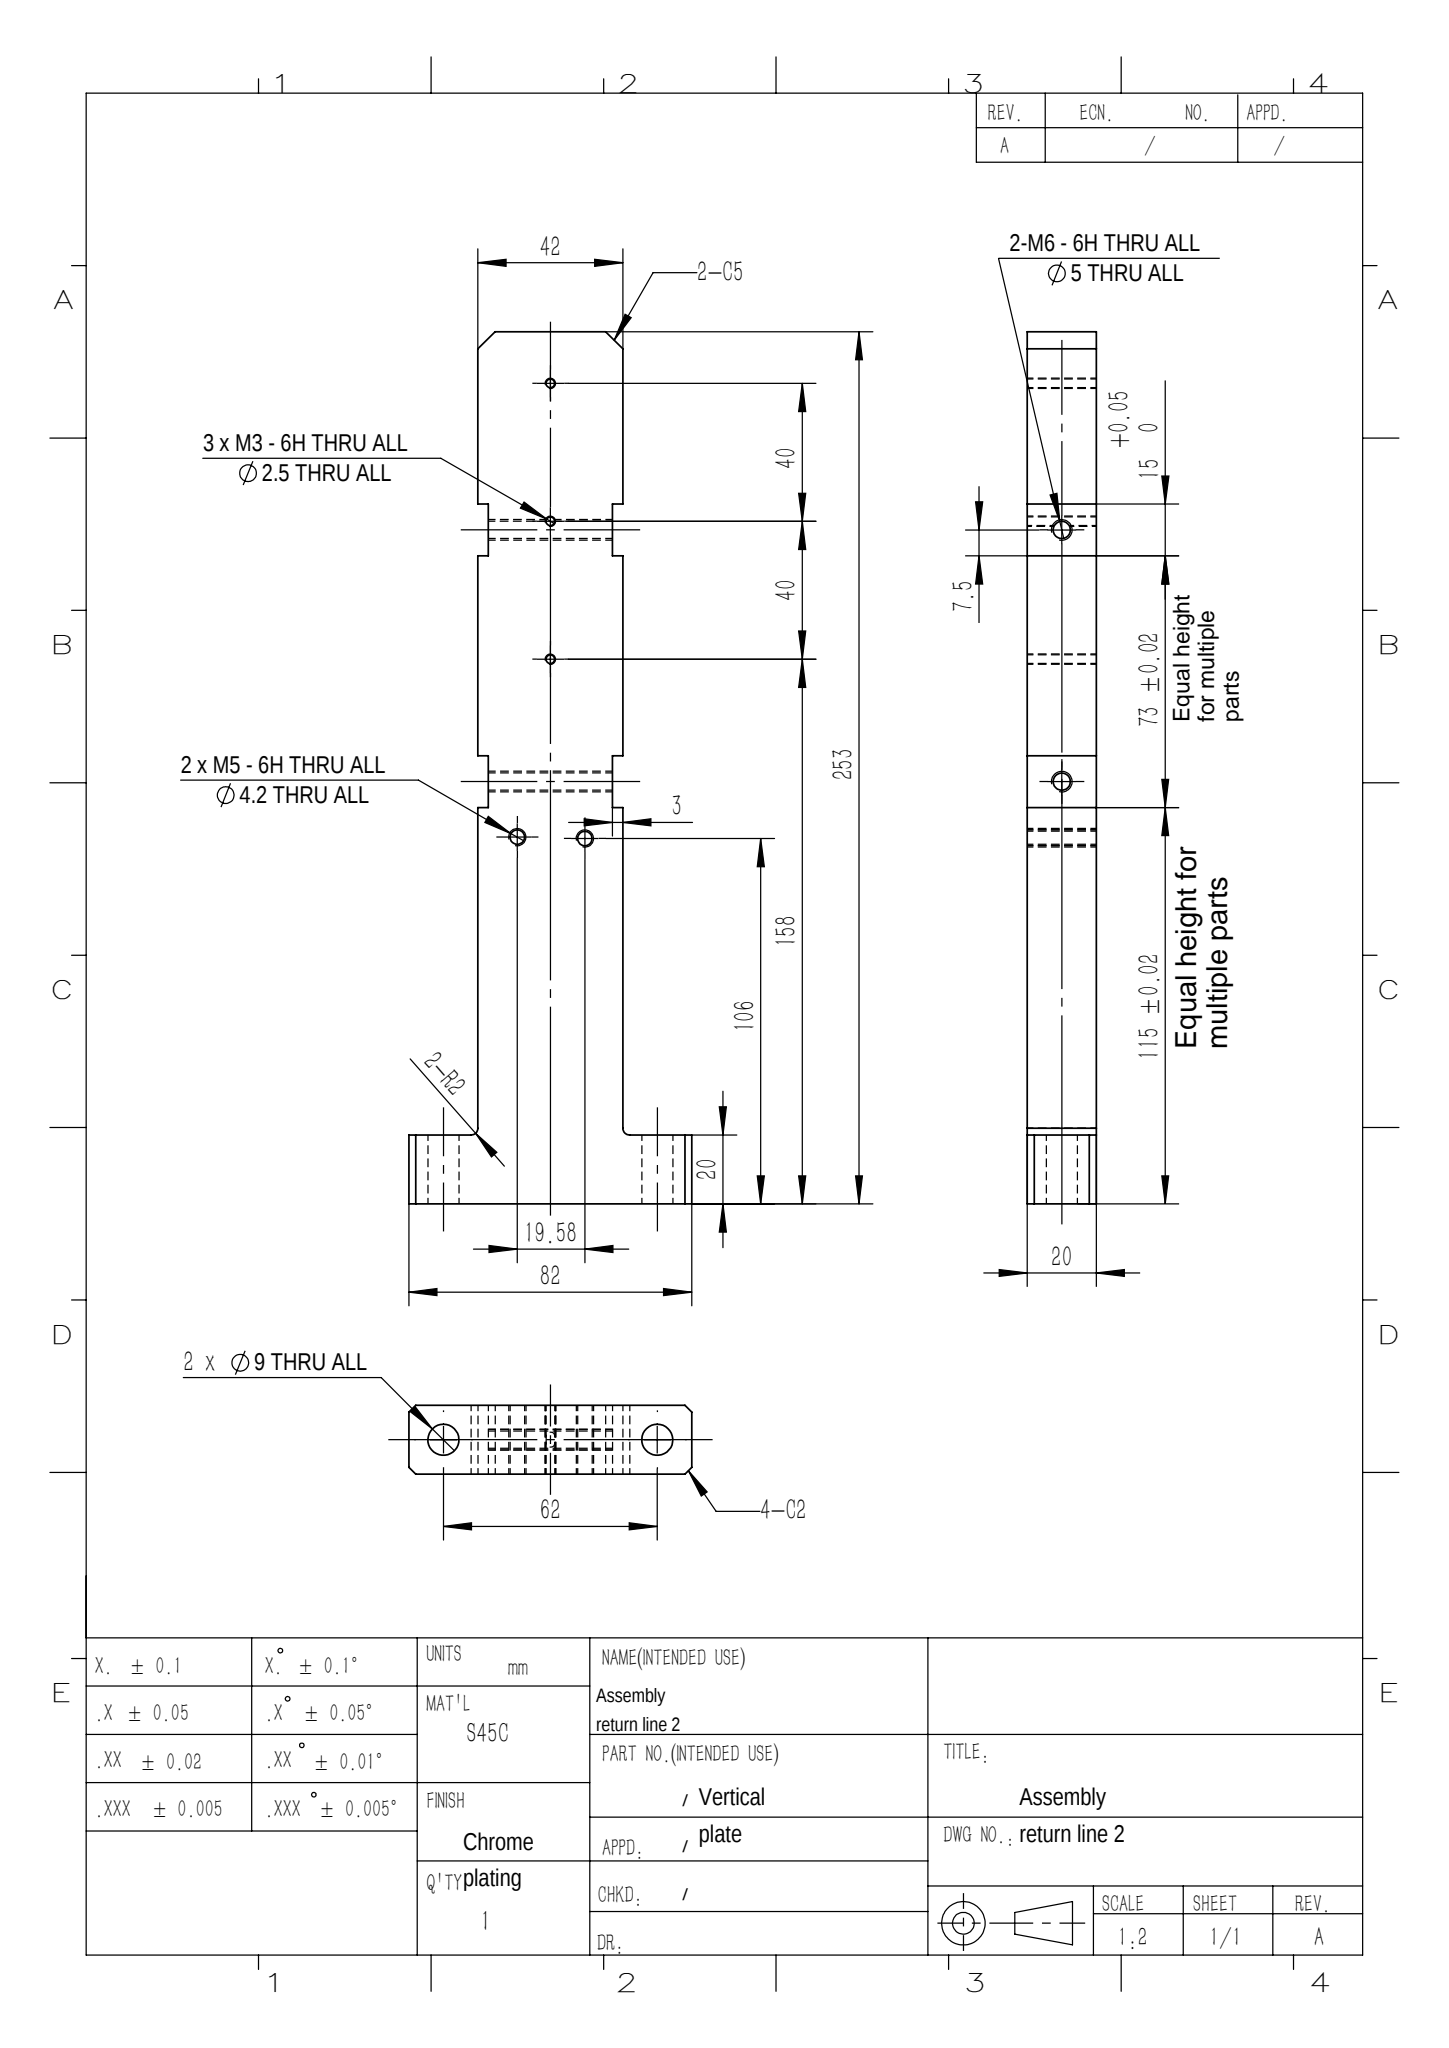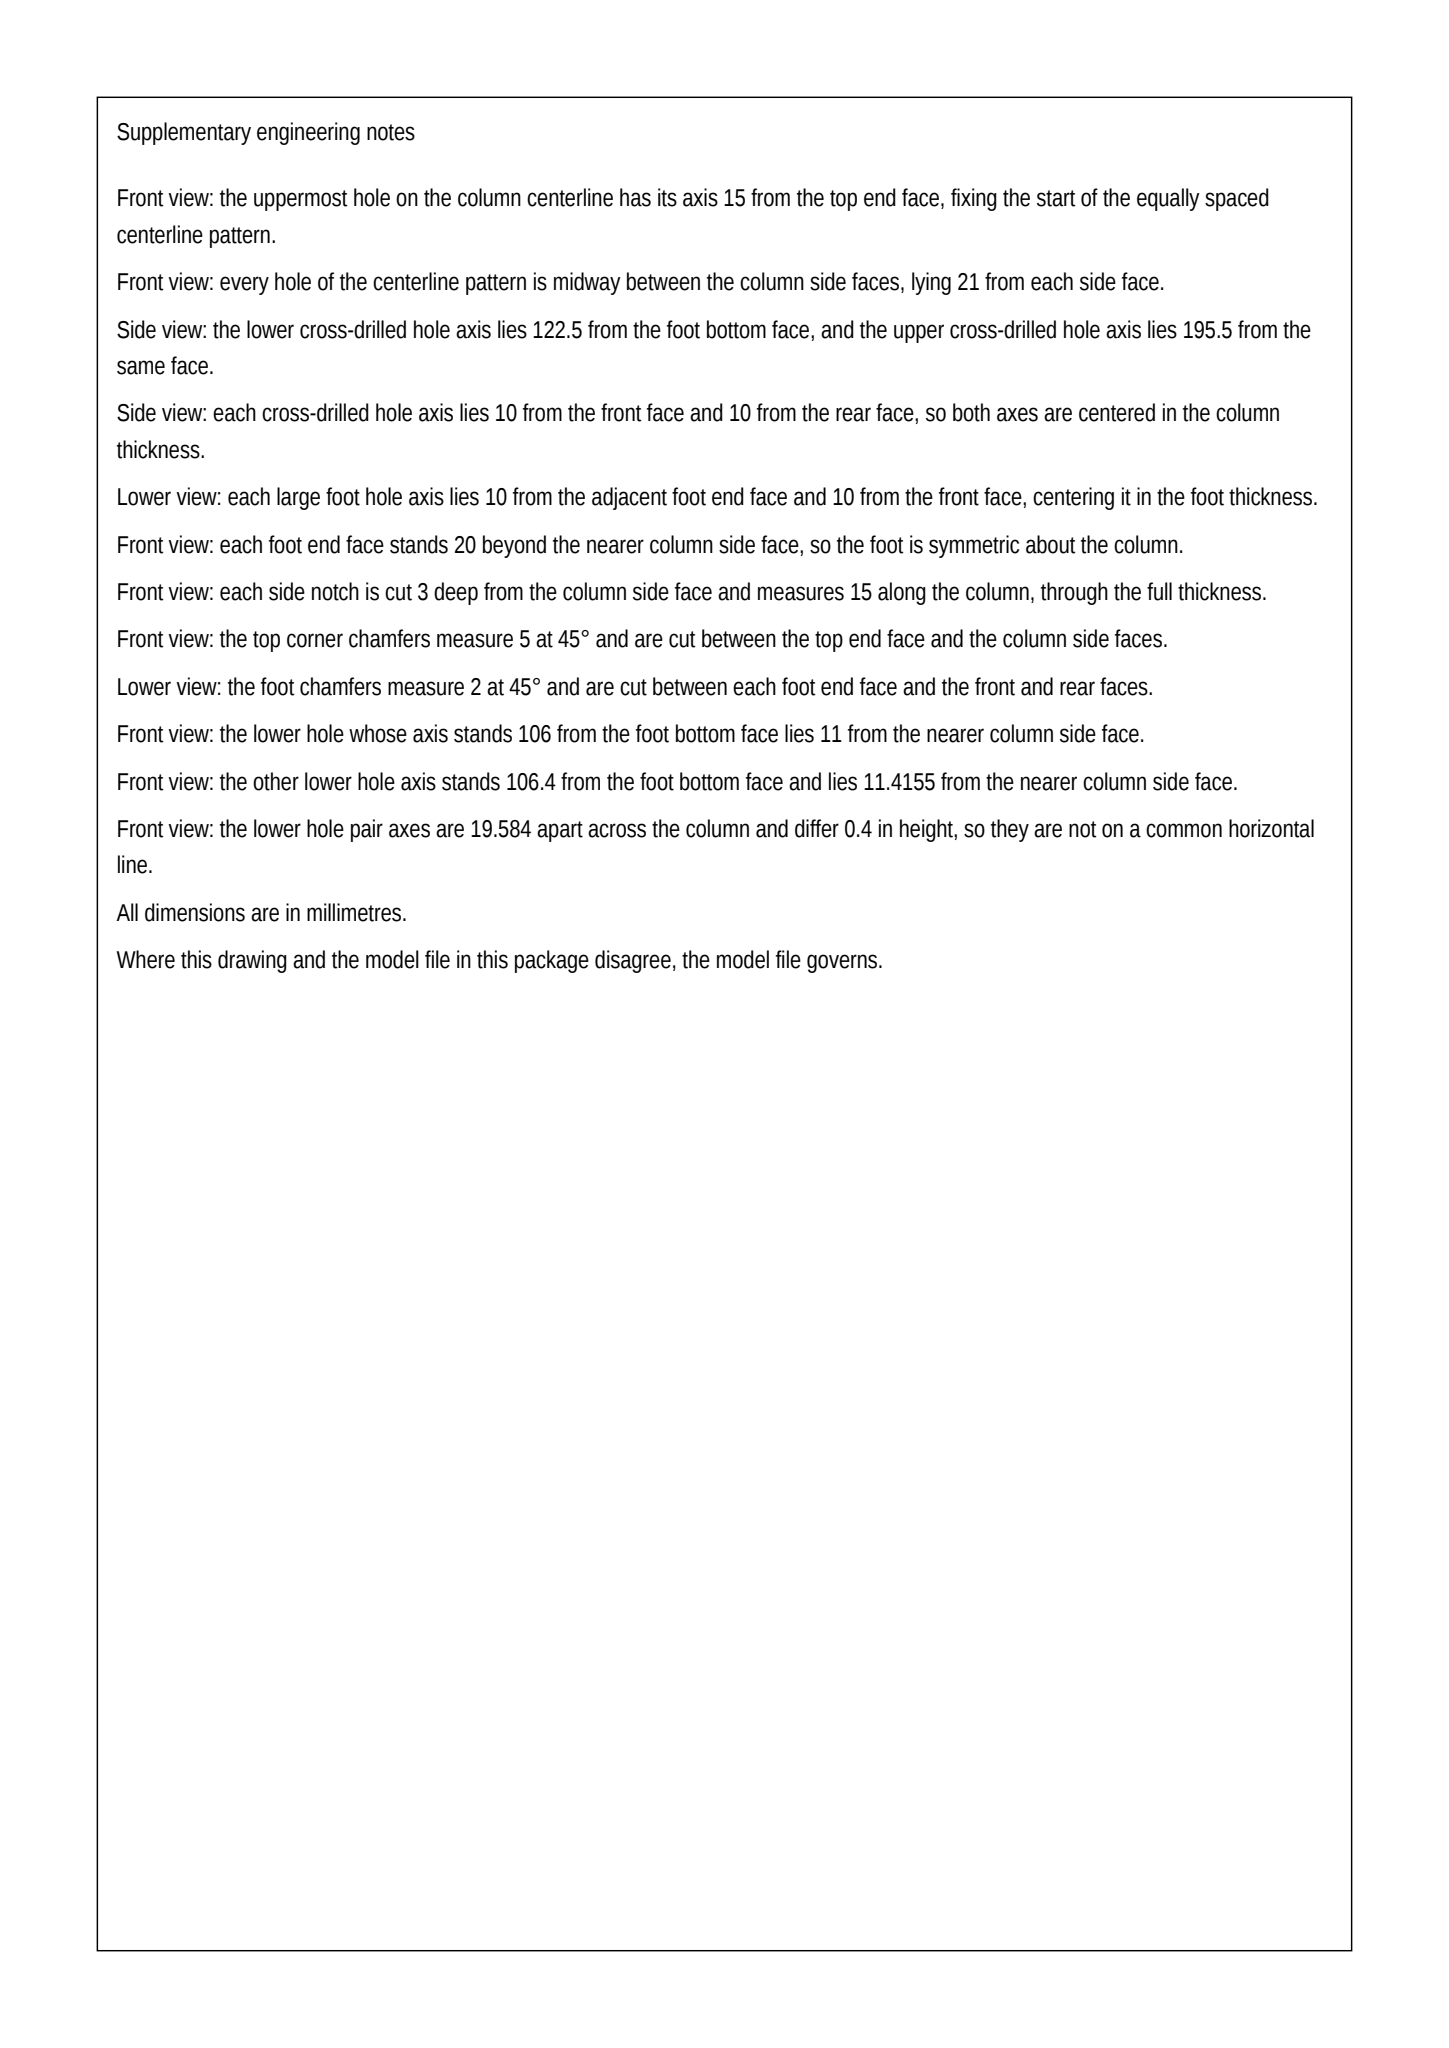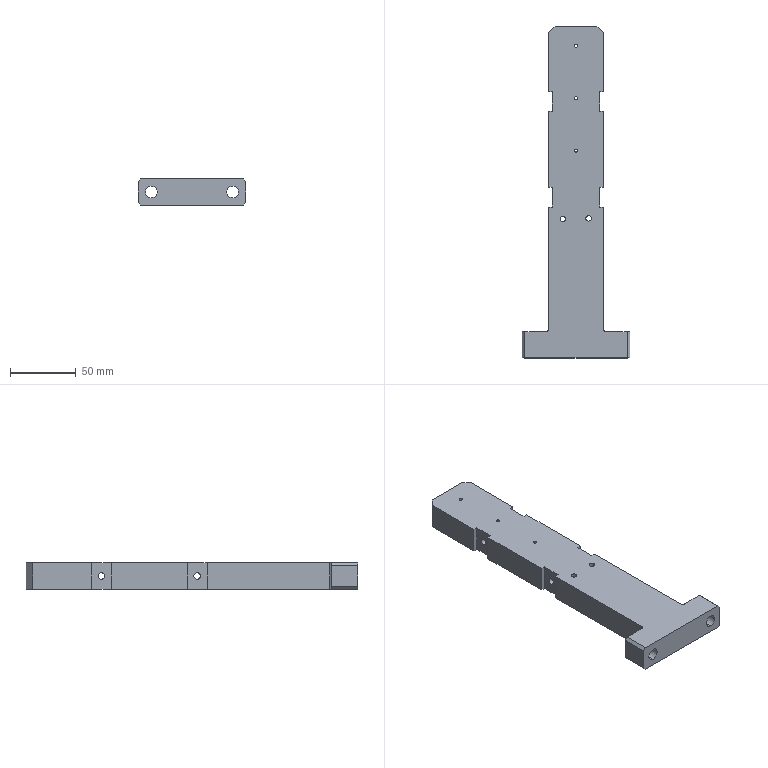Part | SolidWorks | mm | 1 solid | 53 faces | box 82 x 253 x 20 mm | volume 219494 mm3 | plane 32 | cylinder 21 | commonest cylinder face diameters 2.5 x7 5 x4 4.2 x4 9 x4 4 x2
build123d program:
from build123d import *

# Parameters (mm, degrees)
BOSS_EXTRUDE1_DEPTH      = 20
SKETCH2_W                = 3
SKETCH2_H                = 15
CUT_EXTRUDE1_DEPTH       = 20
F_9_0_9_DIAMETER_HOLE1_D = 9
M6_TAPPED_HOLE1_D        = 5
M5_TAPPED_HOLE1_D        = 4.2
M3_TAPPED_HOLE1_D        = 2.5
CHAMFER1_SIZE            = 2
FILLET1_R                = 2
CHAMFER2_SIZE            = 5
M6_TAPPED_HOLE2_D        = 5


with BuildPart() as part:
    # Sketch1 → Boss-Extrude1 (new body)
    with BuildSketch(Plane.XY):
        Polygon((-41, 0), (41, 0), (41, 20), (21, 20), (21, 253), (-21, 253), (-21, 20), (-41, 20), align=None)
    extrude(amount=BOSS_EXTRUDE1_DEPTH)

    # Sketch2 → Cut-Extrude1 (cut)
    with BuildSketch(Plane.XY.offset(20)):
        with Locations((-19.5, 195.5)):
            Rectangle(SKETCH2_W, SKETCH2_H)
        with Locations((19.5, 195.5)):
            Rectangle(SKETCH2_W, SKETCH2_H)
        with Locations((-19.5, 122.5)):
            Rectangle(SKETCH2_W, SKETCH2_H)
        with Locations((19.5, 122.5)):
            Rectangle(SKETCH2_W, SKETCH2_H)
    extrude(amount=-CUT_EXTRUDE1_DEPTH, mode=Mode.SUBTRACT)

    # 9.0 _9_ Diameter Hole1 (through all)
    with Locations(Plane(origin=(0, 0, 0), x_dir=(-1, 0, 0), z_dir=(0, -1, 0))):
        with Locations((31, -10), (-31, -10)):
            Hole(F_9_0_9_DIAMETER_HOLE1_D / 2)

    # M6 Tapped Hole1 (through all)
    with Locations(Plane(origin=(18, 0, 0), x_dir=(0, 0, -1), z_dir=(1, 0, 0))):
        with Locations((-10, 195.5)):
            Hole(M6_TAPPED_HOLE1_D / 2)

    # M5 Tapped Hole1 (through all)
    with Locations(Plane.XY.offset(20)):
        with Locations((9.584, 106.4), (-10, 106)):
            Hole(M5_TAPPED_HOLE1_D / 2)

    # M3 Tapped Hole1 (through all)
    with Locations(Plane.XY.offset(20)):
        with Locations((0, 238), (0, 198), (0, 158)):
            Hole(M3_TAPPED_HOLE1_D / 2)

    # Chamfer1
    chamfer1_edges = [part.edges().sort_by_distance(p)[0] for p in [
        (41, 10, 0),
        (-41, 10, 20),
        (41, 10, 20),
        (-41, 10, 0),
    ]]
    chamfer(chamfer1_edges, length=CHAMFER1_SIZE)

    # Fillet1
    fillet1_edges = [part.edges().sort_by_distance(p)[0] for p in [
        (-21, 20, 10),
        (21, 20, 10),
    ]]
    fillet(fillet1_edges, radius=FILLET1_R)

    # Chamfer2
    chamfer2_edges = [part.edges().sort_by_distance(p)[0] for p in [
        (-21, 253, 10),
        (21, 253, 10),
    ]]
    chamfer(chamfer2_edges, length=CHAMFER2_SIZE)

    # M6 Tapped Hole2 (through all)
    with Locations(Plane.ZY.offset(18)):
        with Locations((10, 122.5)):
            Hole(M6_TAPPED_HOLE2_D / 2)


solid = part.part